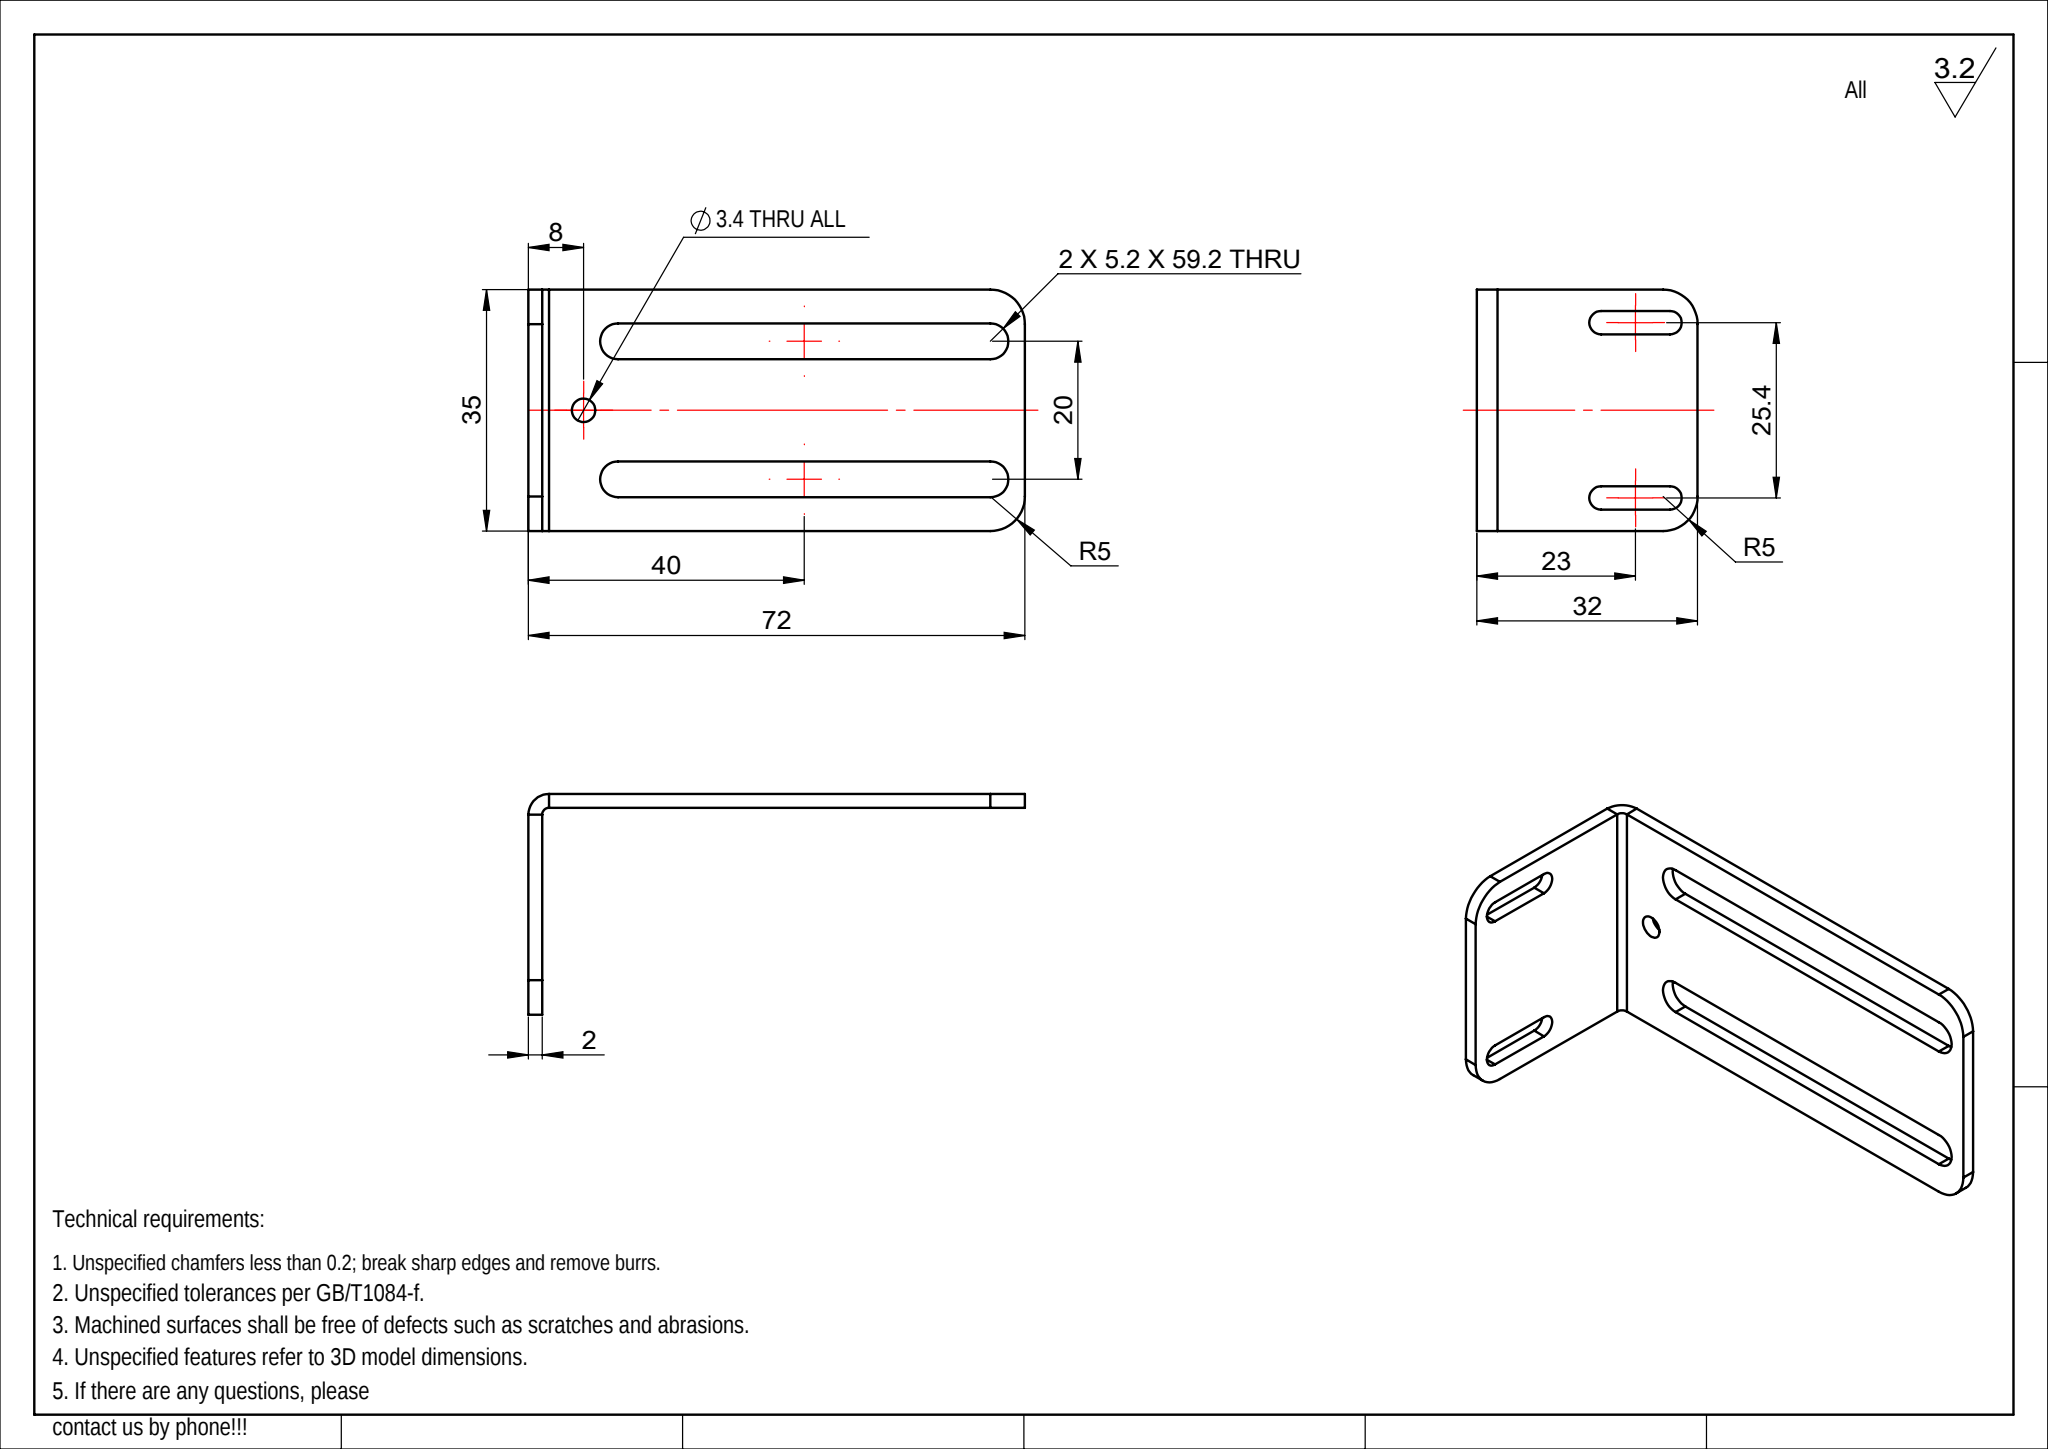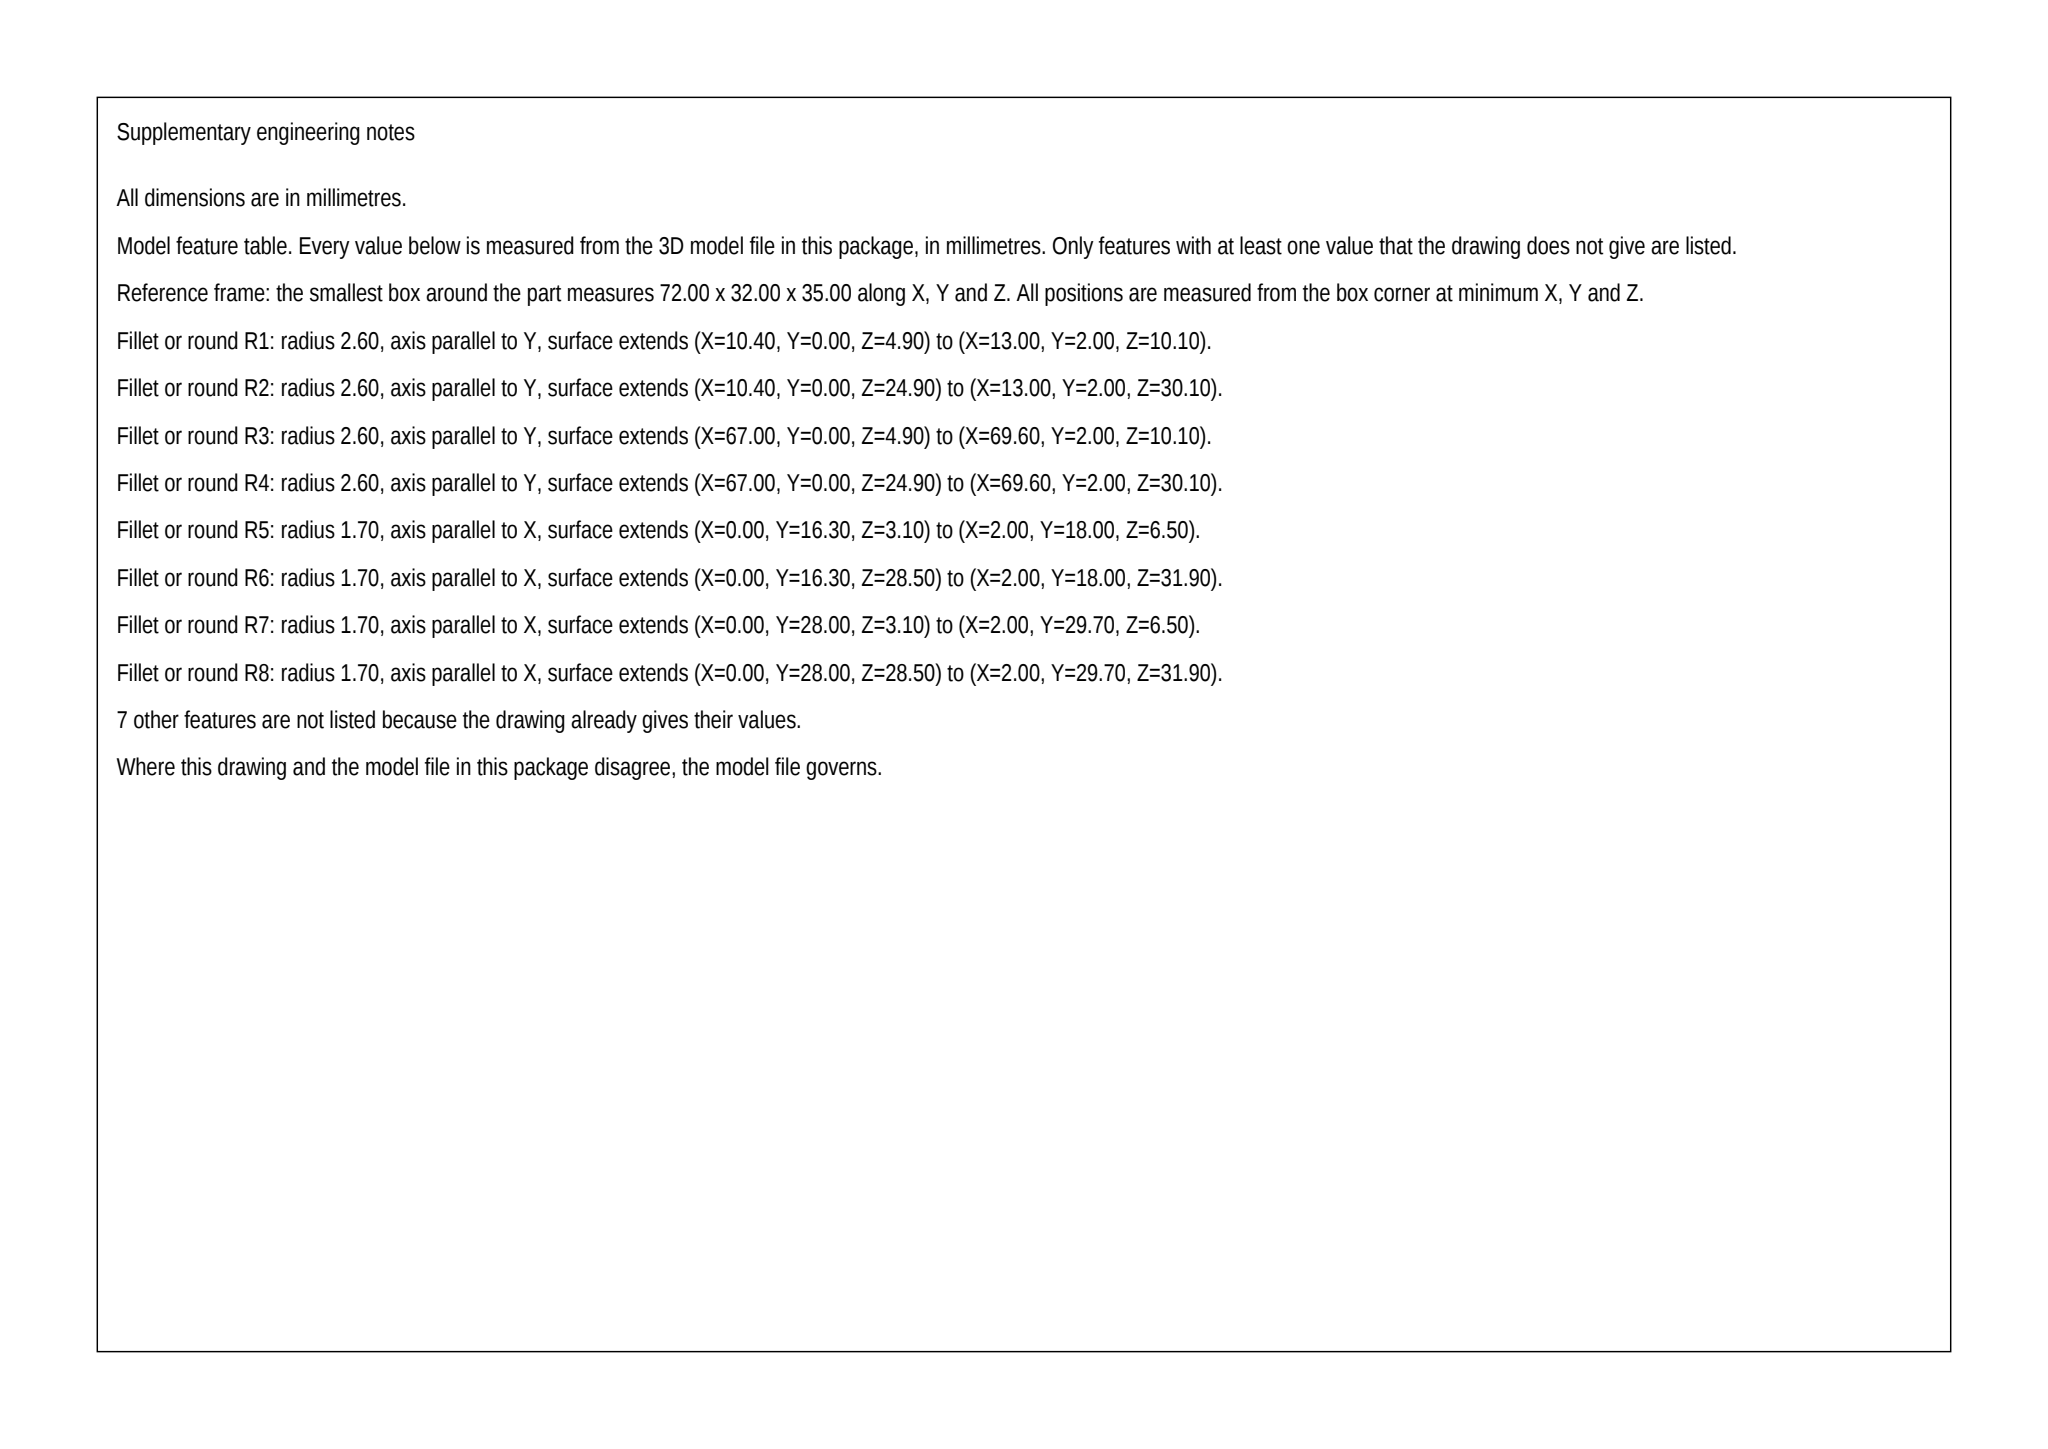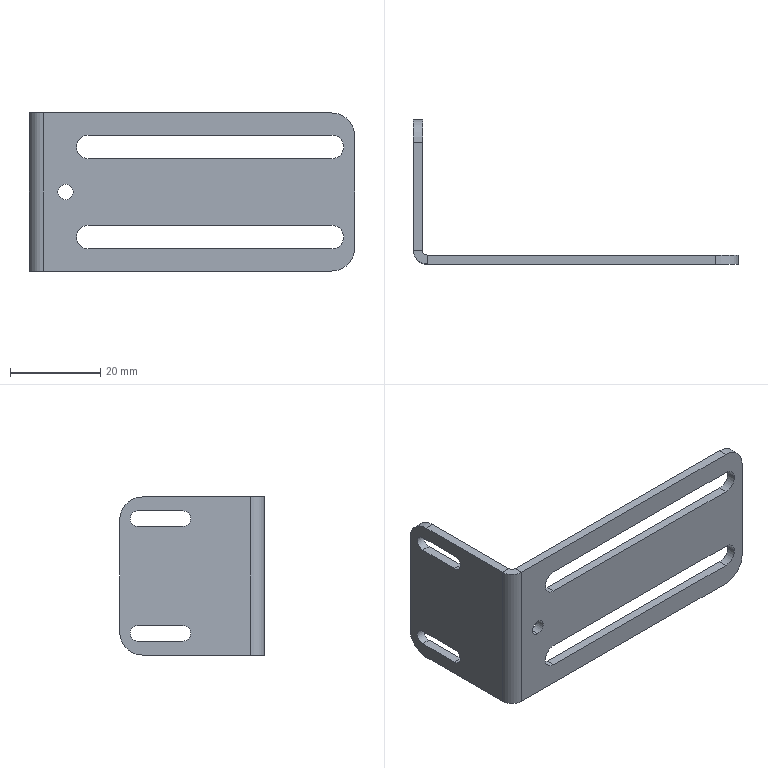Part | SolidWorks | mm | 1 solid | 38 faces | box 72 x 32 x 35 mm | volume 5638 mm3 | plane 20 | cylinder 18 | commonest cylinder face diameters 3.4 x6 5.2 x6 10 x4 6 x1 2 x1